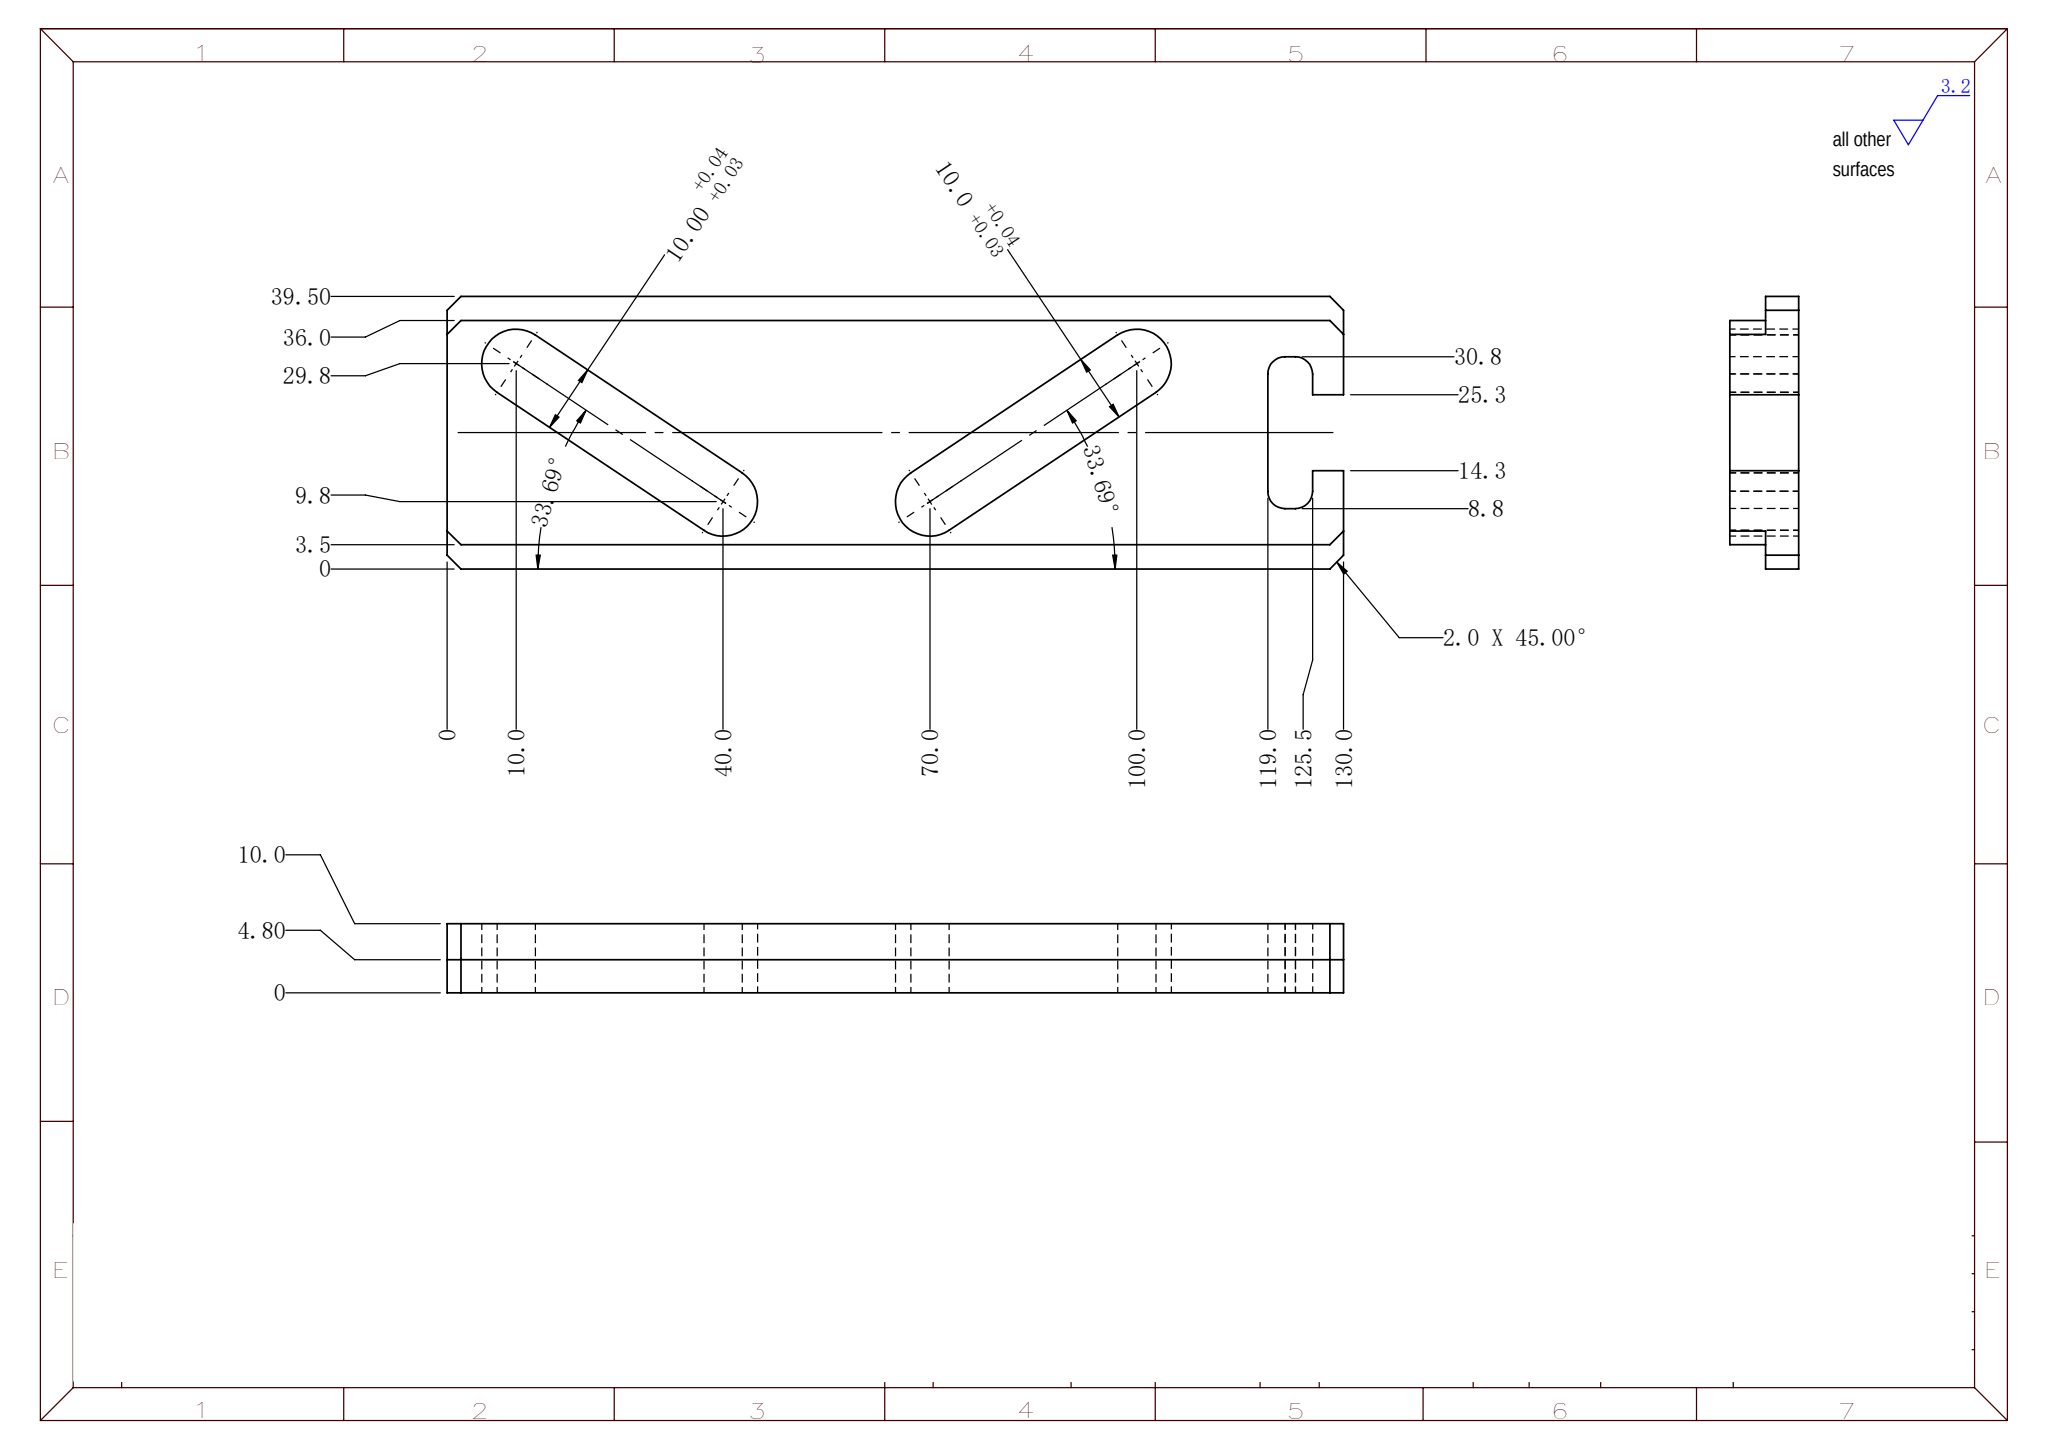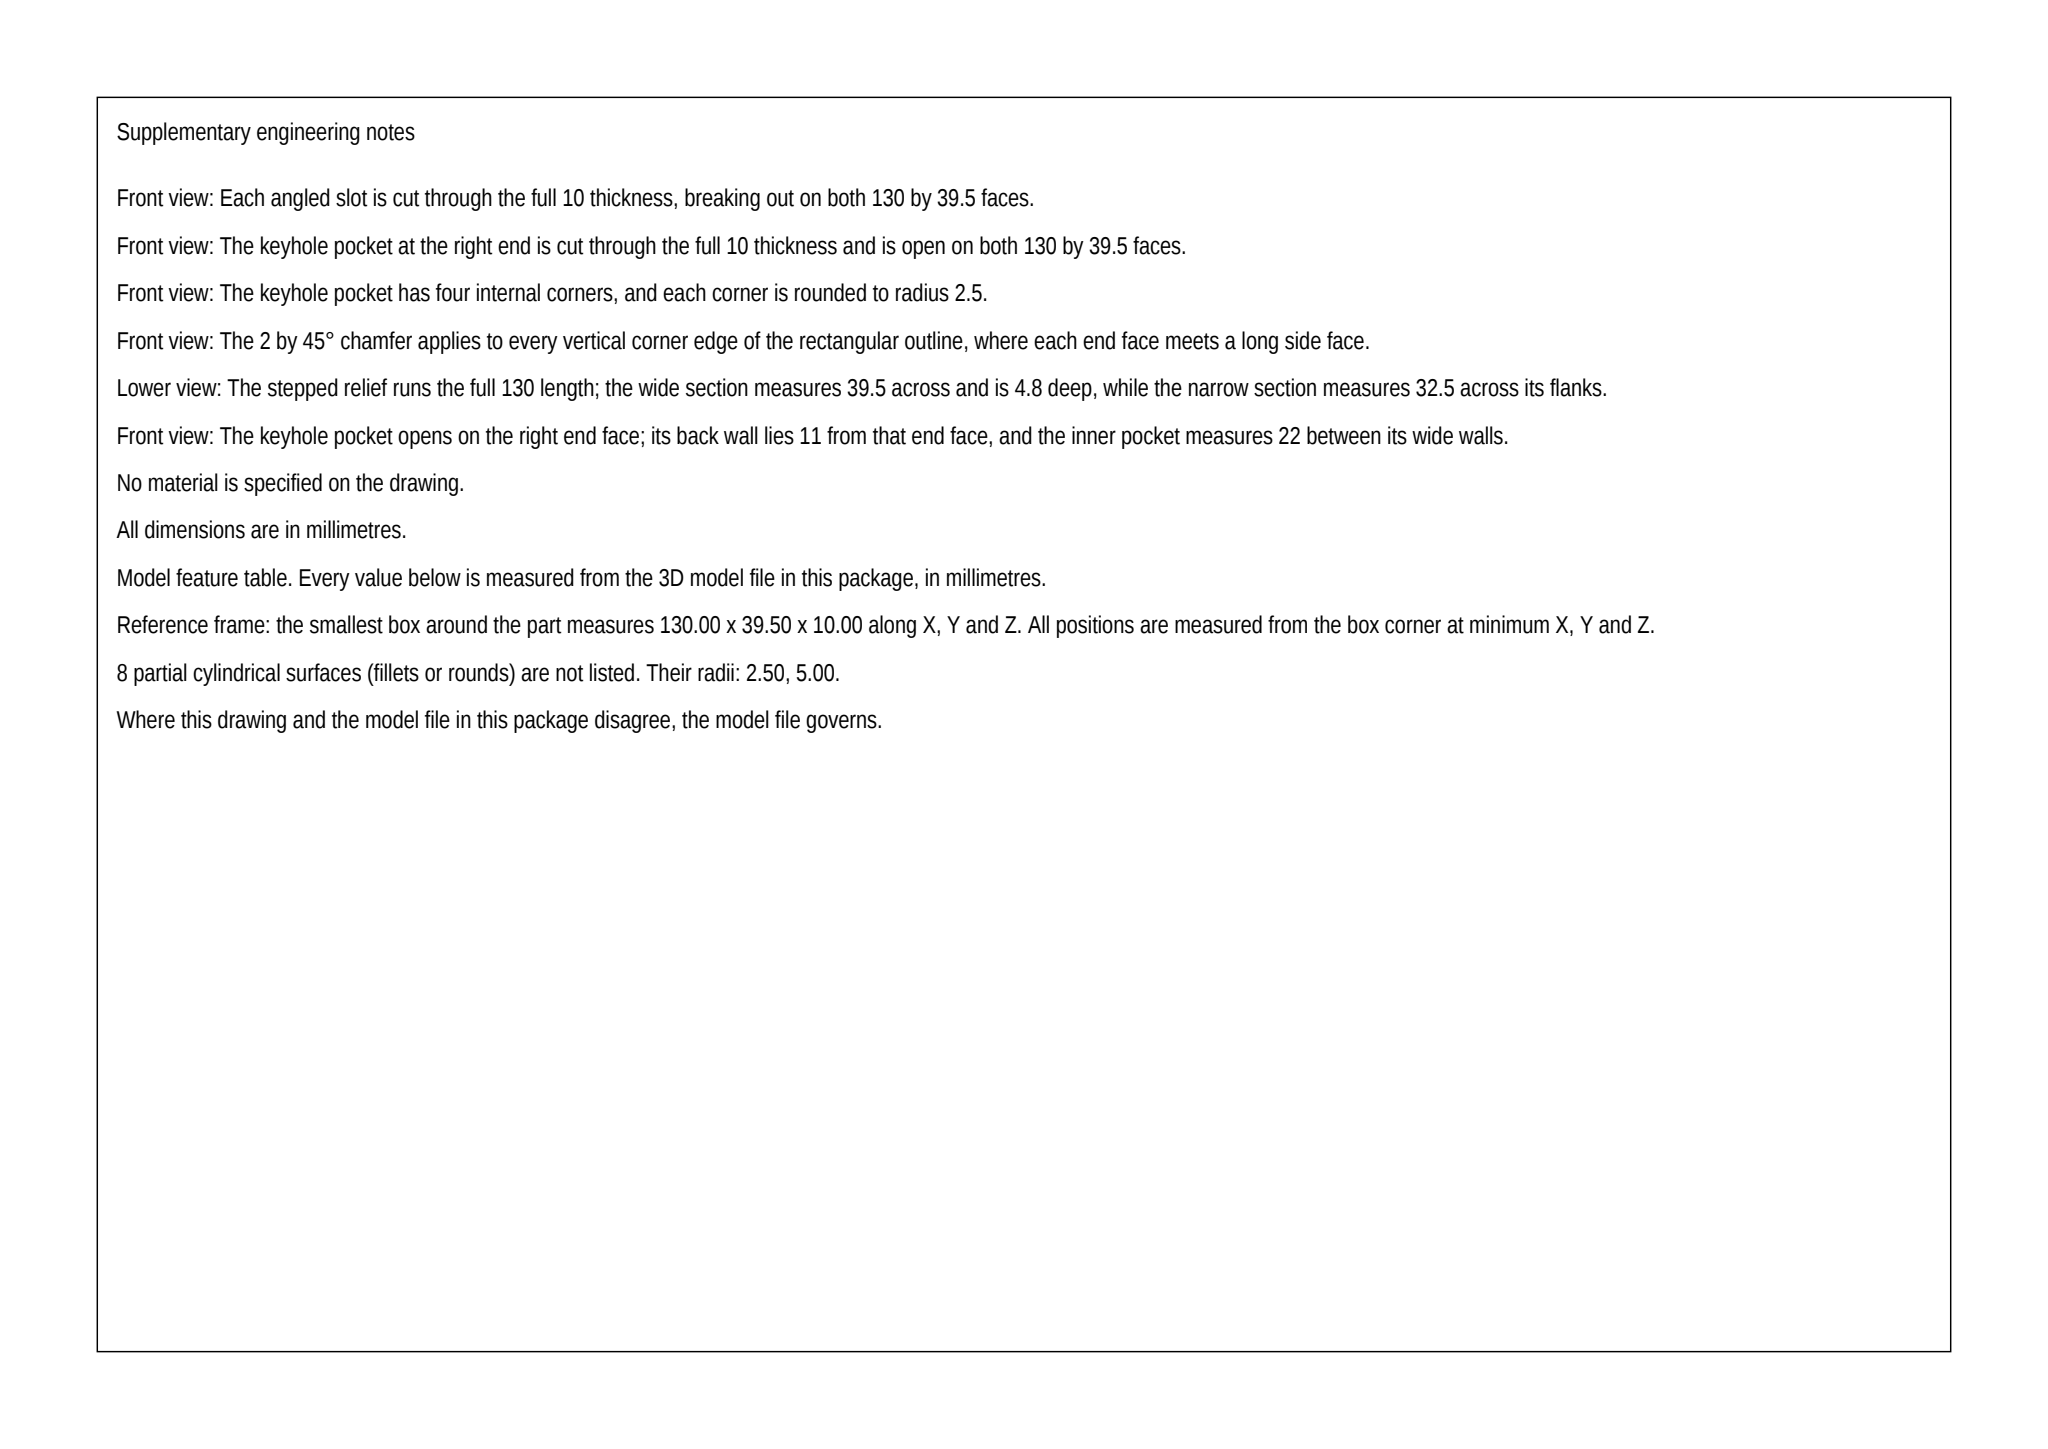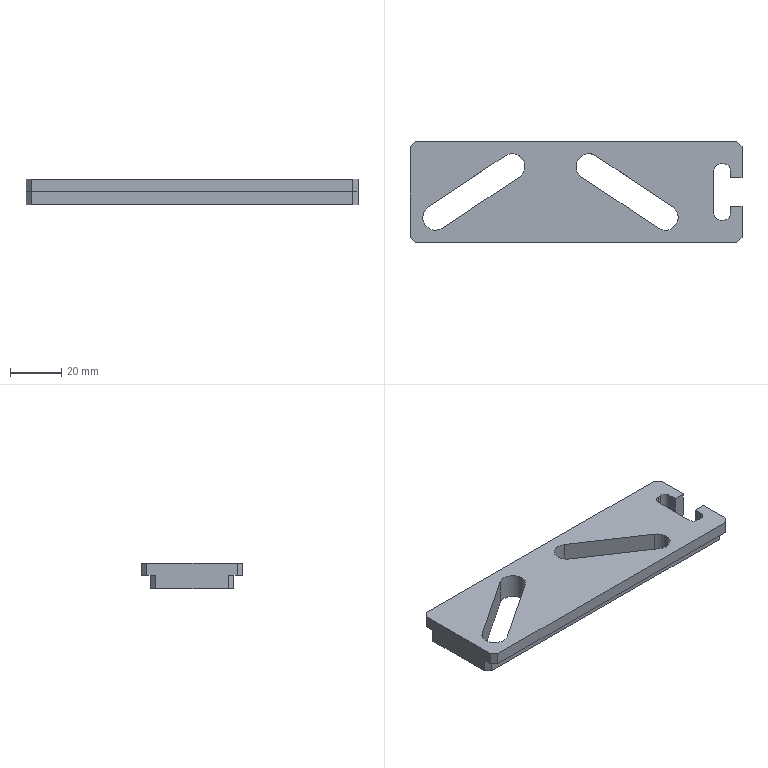Part | SolidWorks | mm | 1 solid | 40 faces | box 130 x 39.5 x 10 mm | volume 35885 mm3 | plane 30 | cylinder 10 | commonest cylinder face diameters 10 x6 5 x4
Drawing notes:
2X CHAM 3.5 X 45.00° AT LH END CORNERS (TOP VIEW) | from the solid: X=0 end face lies between Y=3.5 and Y=36.0 planes, outer edges Y=0/Y=39.5 -> 3.5 leg each way at 45 deg
2.0 X 45.00° TYP BOTH RH CORNERS - PART SYMM ABOUT CL | from the solid: Y planes 0/39.5, 3.5/36.0, 8.75/30.75, 14.25/25.25 and slots Y=9.75/29.75 all mirror about Y=19.75
SIDE STEP 4.8 DEEP FROM TOP FACE; STEP FACE 5.2 ABOVE BOTTOM | from the solid: Z planes 0, 5.2 (2 faces), 10.0; bbox Z=10.0 -> 10.0-5.2=4.8
UNLESS OTHERWISE SPECIFIED ALL DIMS IN MM | from the solid: STEP model units mm; bbox 130.0 x 39.5 x 10.0 mm